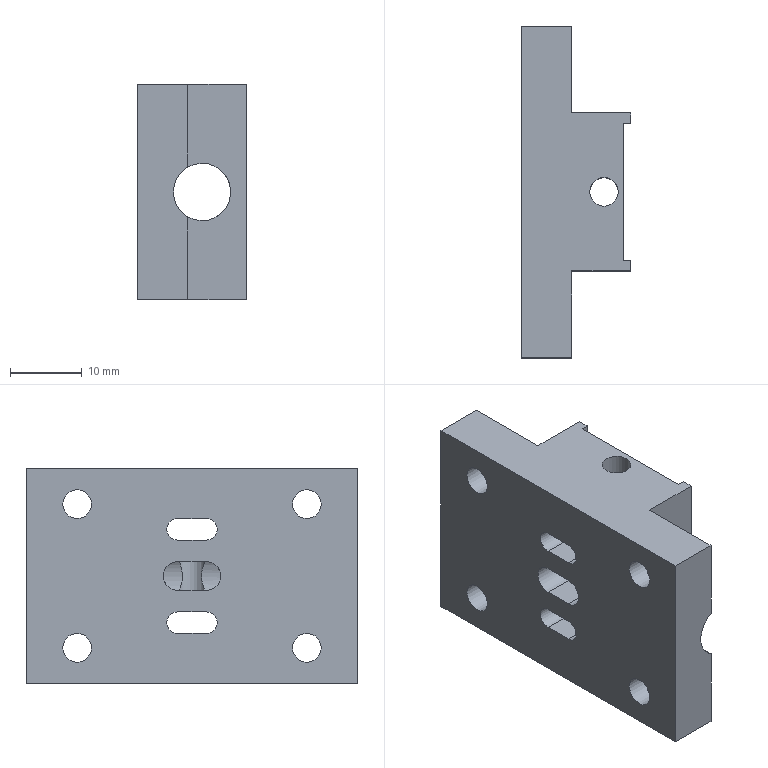Component | NX | 03D__27_2 | 1 solid | 40 faces | volume 11928 mm3 | plane 26 | cylinder 14 | commonest cylinder face diameters 4 x9 3 x4 8 x1